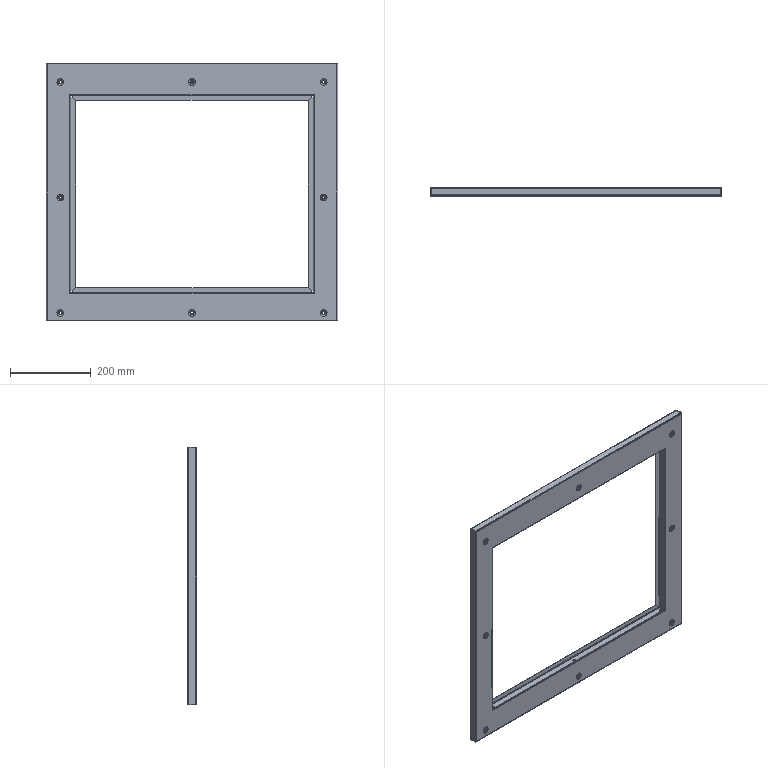Component | SolidWorks | 01-12RearGuardPlate-1 | 1 solid | 322 faces | volume 465900 mm3 | plane 106 | cylinder 96 | torus 64 | spline 56 | commonest cylinder face diameters 15 x16 12 x16 6.5 x16 7 x12 2 x12 4.473 x8 1.473 x8 5 x8 | material SPCC